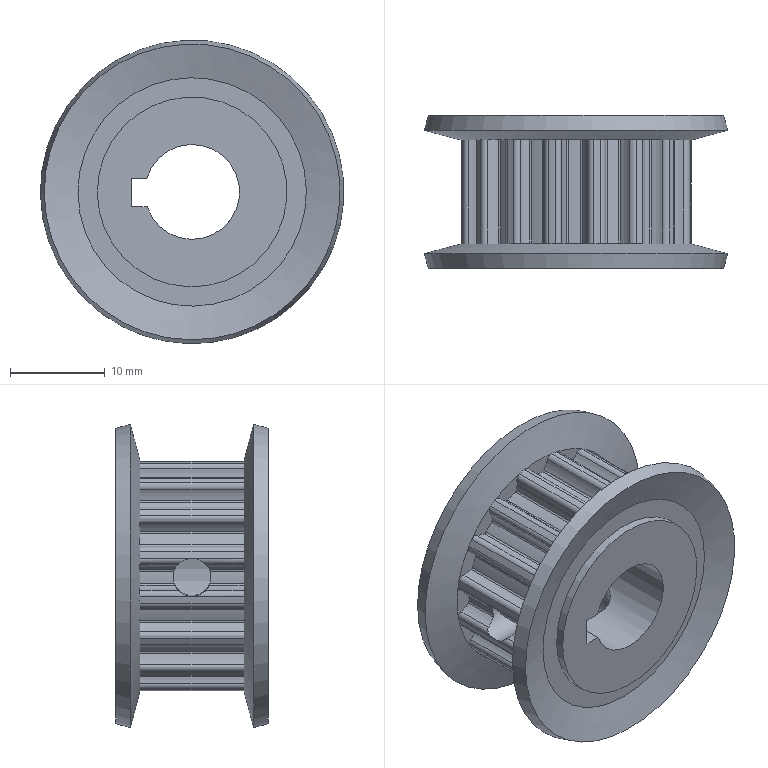Component | NX | SYNCHRONOUS_PULLEY_1 | 1 solid | 193 faces | volume 6050 mm3 | cylinder 145 | plane 42 | cone 6 | commonest cylinder face diameters 6.55 x36 0.5 x35 1.1 x34 20.96 x18 24.5 x17 20 x2 4 x2 10 x1